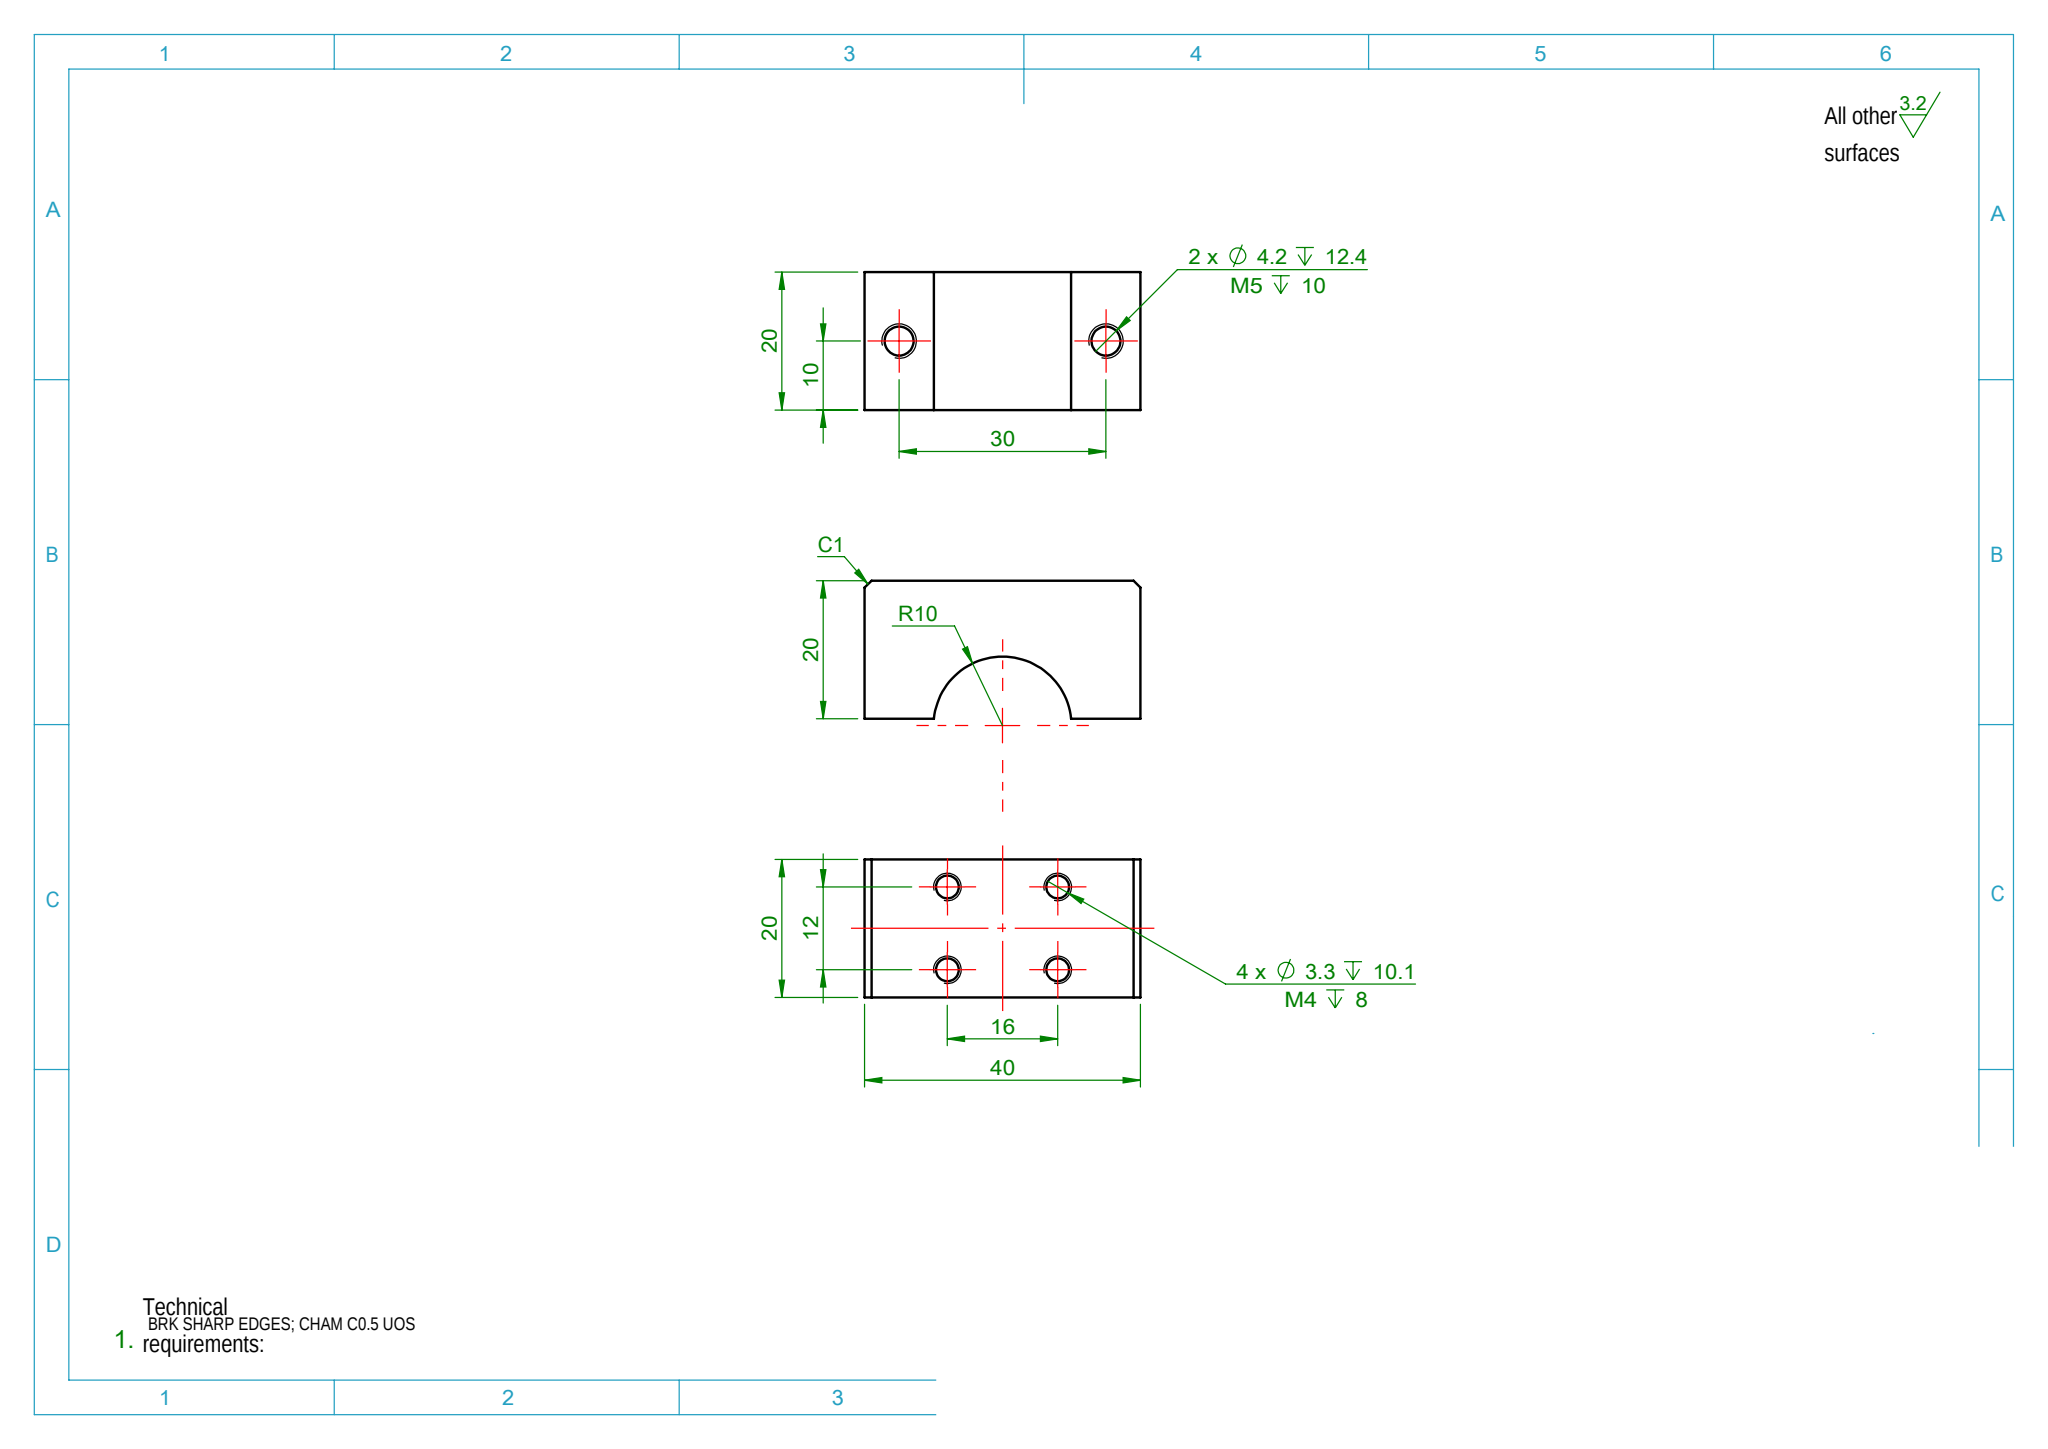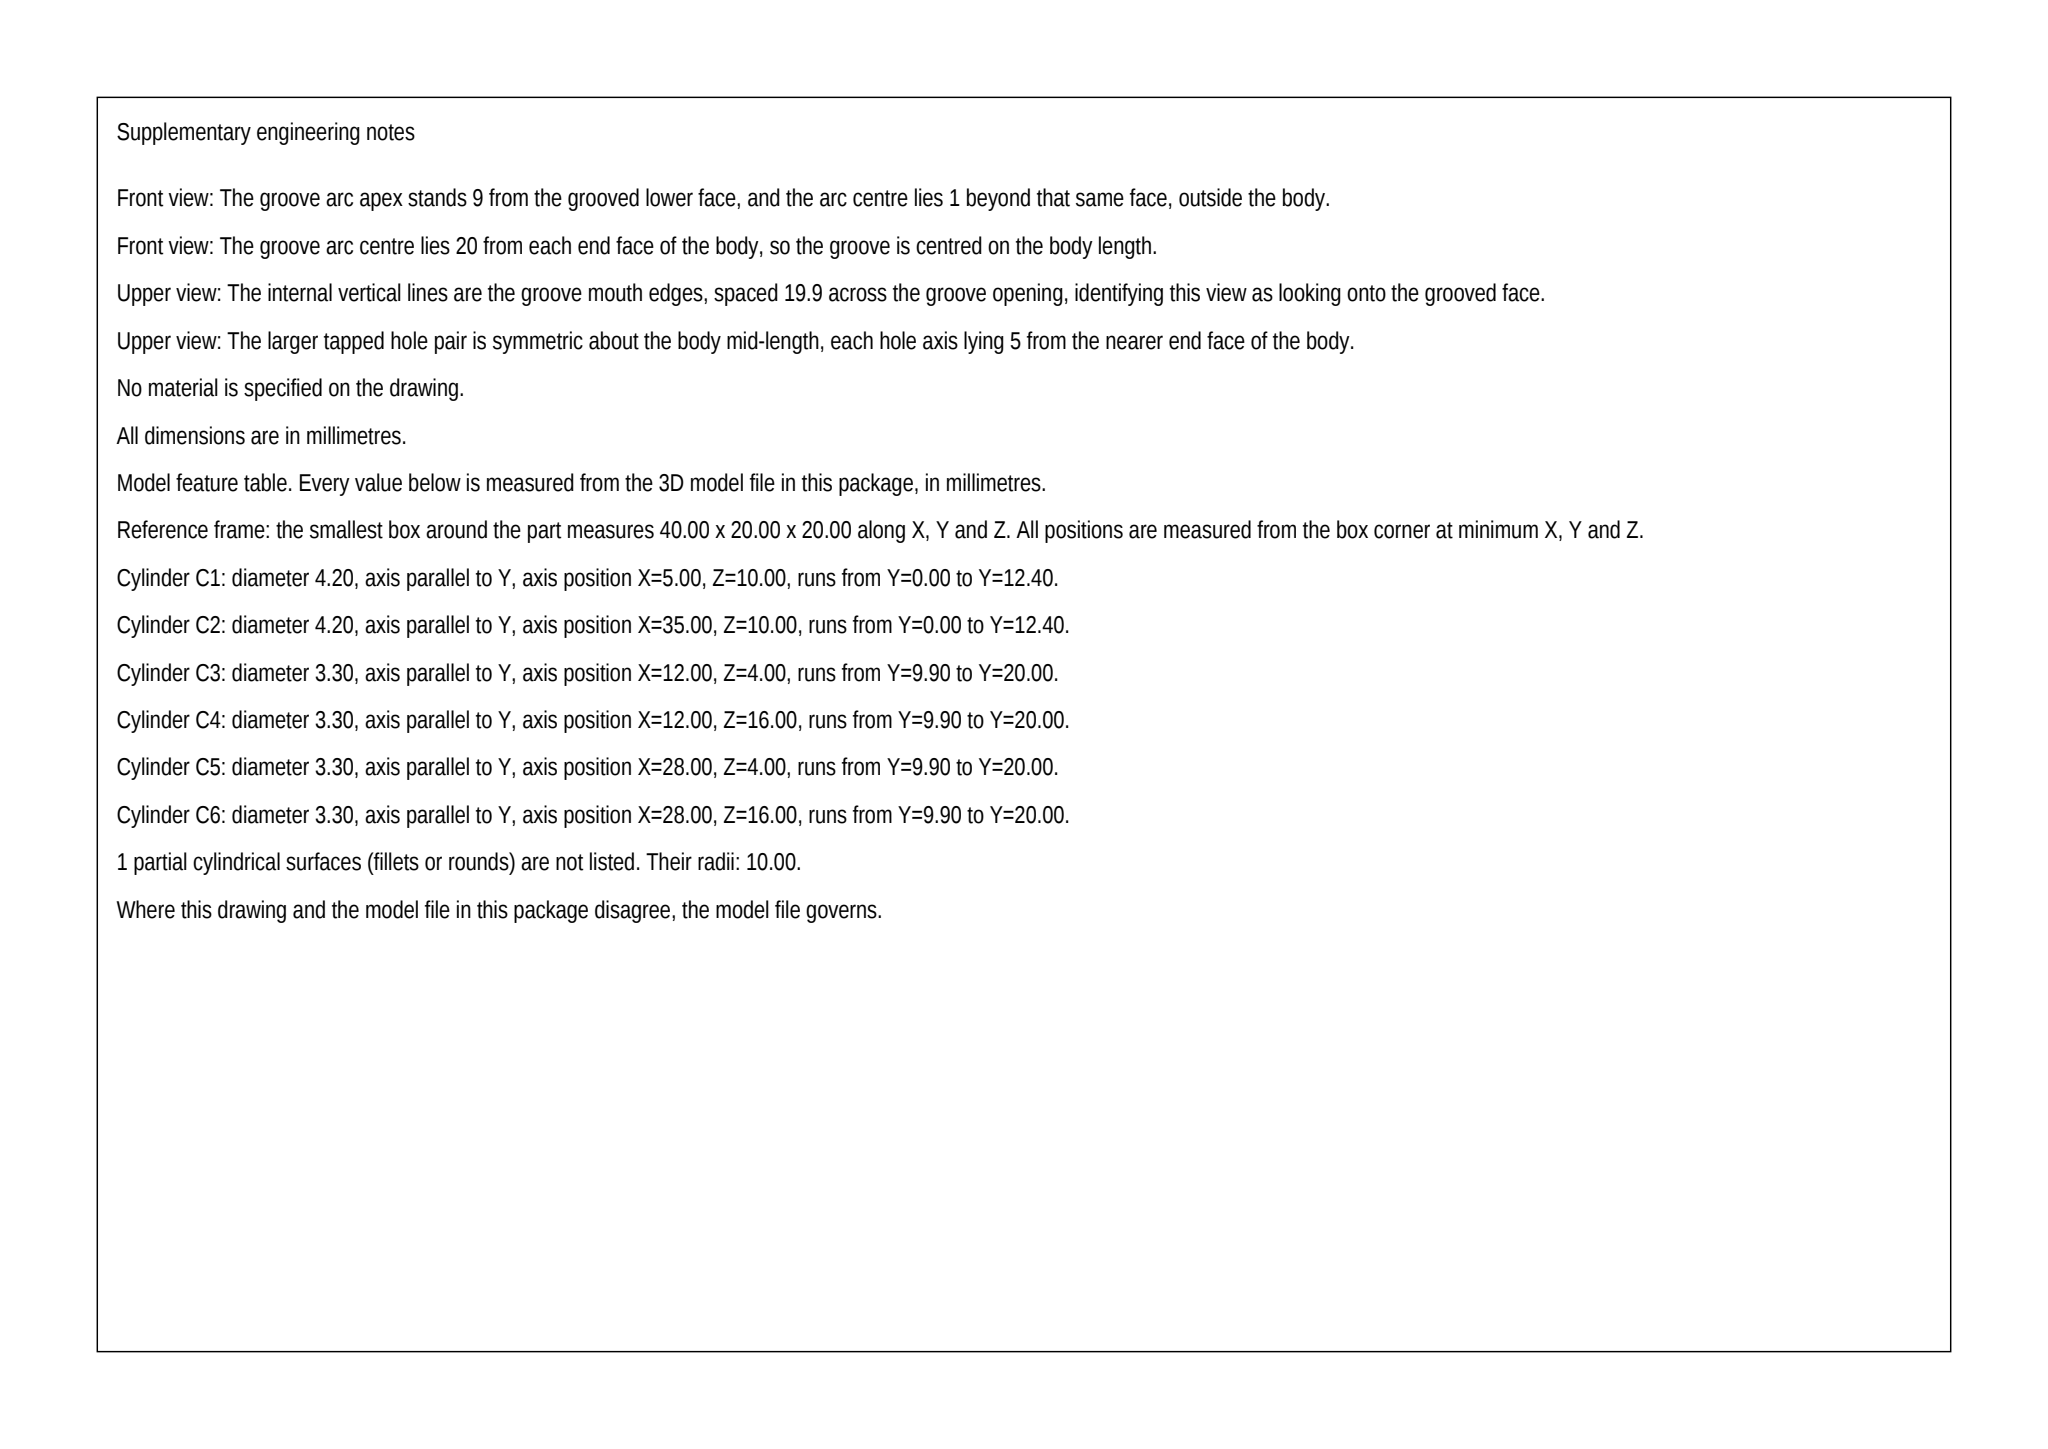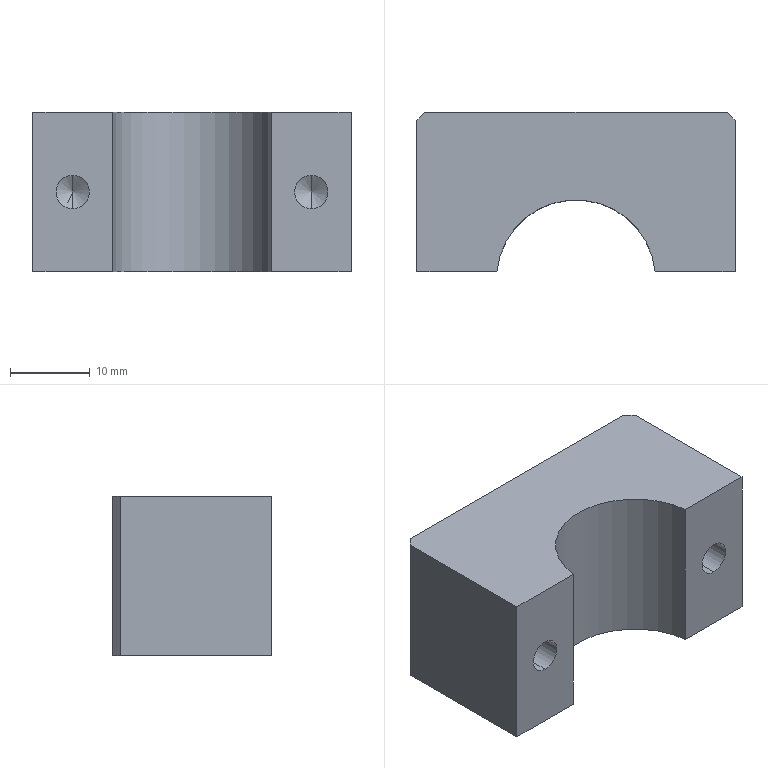Part | SolidWorks | mm | 1 solid | 34 faces | box 40 x 20 x 20 mm | volume 12526 mm3 | cylinder 13 | cone 12 | plane 9 | commonest cylinder face diameters 3.3 x8 4.2 x4 20 x1
Drawing notes:
R10 NOTCH: ARC CL 1 BELOW BOTTOM FACE, NOTCH DEPTH 9 | from the solid: cylinder dia 20, axis z, pos (x=20.0, y=-1.0); bbox y 0..20 so arc center 1 mm below bottom face, cut depth = 10-1 = 9
build123d program:
from build123d import *

# Parameters (mm, degrees)
SKETCH1_W             = 40
SKETCH1_H             = 20
BOSS_EXTRUDE1_DEPTH   = 20
SKETCH2_R             = 10
CUT_EXTRUDE1_DEPTH    = 31
CHAMFER1_SIZE         = 1
M5_TAPPED_HOLE1_D     = 4.2
M5_TAPPED_HOLE1_DEPTH = 12.4
M5_TAPPED_HOLE1_TIP   = 1.262
M4_TAPPED_HOLE1_D     = 3.3
M4_TAPPED_HOLE1_DEPTH = 10.1
M4_TAPPED_HOLE1_TIP   = 0.9914


with BuildPart() as part:
    # Sketch1 → Boss-Extrude1 (new body)
    with BuildSketch(Plane.XY):
        Rectangle(SKETCH1_W, SKETCH1_H)
    extrude(amount=BOSS_EXTRUDE1_DEPTH)

    # Sketch2 → Cut-Extrude1 (cut, through all)
    with BuildSketch(Plane.XY.offset(20)):
        with Locations((0, -11)):
            Circle(SKETCH2_R)
    extrude(amount=-CUT_EXTRUDE1_DEPTH, mode=Mode.SUBTRACT)

    # Chamfer1
    chamfer1_edges = [part.edges().sort_by_distance(p)[0] for p in [
        (-20, 10, 10),
        (20, 10, 10),
    ]]
    chamfer(chamfer1_edges, length=CHAMFER1_SIZE)

    # M5 Tapped Hole1
    with Locations(Plane(origin=(0, -10, 0), x_dir=(-1, 0, 0), z_dir=(0, -1, 0))):
        with Locations((-15, -10), (15, -10)):
            Hole(M5_TAPPED_HOLE1_D / 2, depth=M5_TAPPED_HOLE1_DEPTH)
            with Locations((0, 0, -(M5_TAPPED_HOLE1_DEPTH + M5_TAPPED_HOLE1_TIP / 2))):  # 118° drill point
                Cone(0, M5_TAPPED_HOLE1_D / 2, M5_TAPPED_HOLE1_TIP, mode=Mode.SUBTRACT)

    # M4 Tapped Hole1
    with Locations(Plane(origin=(0, 10, 0), x_dir=(1, 0, 0), z_dir=(0, 1, 0))):
        with Locations((-8, -16), (-8, -4), (8, -16), (8, -4)):
            Hole(M4_TAPPED_HOLE1_D / 2, depth=M4_TAPPED_HOLE1_DEPTH)
            with Locations((0, 0, -(M4_TAPPED_HOLE1_DEPTH + M4_TAPPED_HOLE1_TIP / 2))):  # 118° drill point
                Cone(0, M4_TAPPED_HOLE1_D / 2, M4_TAPPED_HOLE1_TIP, mode=Mode.SUBTRACT)


solid = part.part